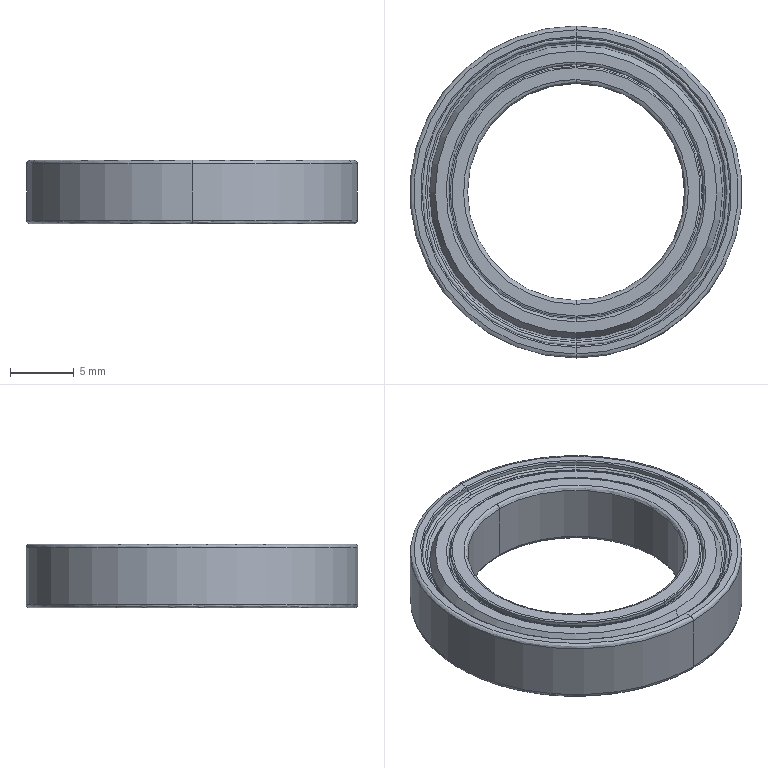Component | SolidWorks | 170423A4-ConveyorSynchronousPulleyAssembly-1_170423A4-BFY01-6803ZZ-L30-1_170423A4-HI_BAY6803ZZ-2 | 1 solid | 137 faces | volume 1172 mm3 | spline 52 | cone 50 | cylinder 24 | plane 11 | commonest cylinder face diameters 24.15 x4 19.95 x4 20.35 x4 20.25 x4 19.65 x4 26 x2 17 x2